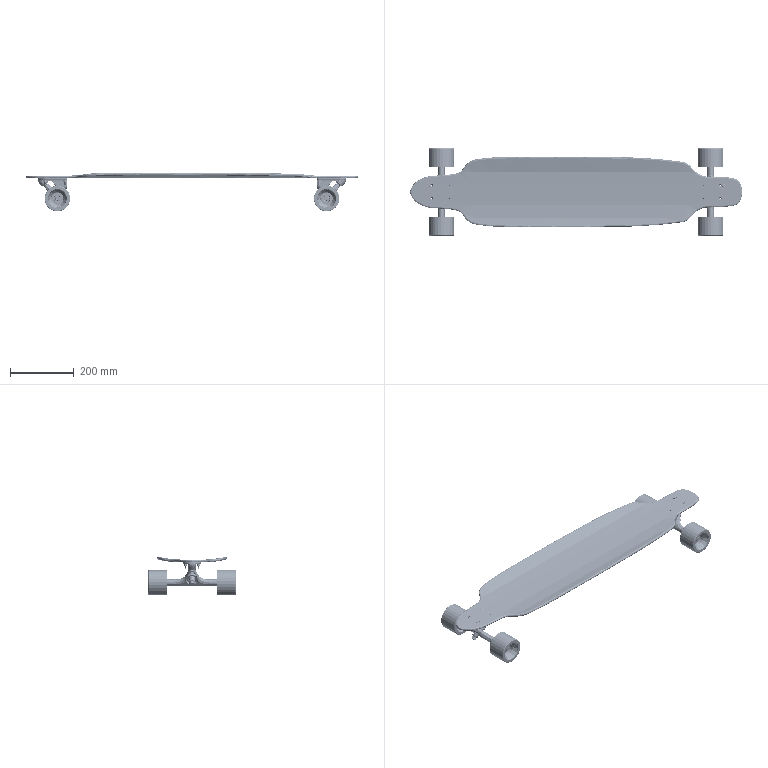Assembly | NX | mm | 63 component files | 63 solids | 1914 faces | box 1041.4 x 274 x 121.11 mm | volume 2752970 mm3 | plane 606 | cylinder 528 | cone 304 | spline 228 | torus 220 | other 20 | sphere 8 | commonest cylinder face diameters 0.26 x96 0.4 x68 0.25 x48 4 x40 6.53 x36 10 x32 5 x32 8 x20
Bill of materials:
unnamed part 1 | 7 |  | Flat circular annular ring (plain washer-like shape) with a central round through-hole and slightly rounded edges.
unnamed part 2 | 8 |  | Countersunk (flat, conical-underside) head screw with a cross-shaped recess in the head and a fully threaded straight shank.
unnamed part 3 | 4 |  | Hex nut with a cylindrical collar on one face. The collar has six radial slots and a raised inner ring around a threaded bore.
unnamed part 4 | 4 |  | Short thick-walled ring with a central bore, rounded edges and concentric annular grooves on the end face, similar in outline to a sealed ball bearing.
unnamed part 5 | 1 |  | Long, thin, flat board with a wide central section that narrows into rounded tabs at both ends. Each tab has a small group of through-holes. The board has a gentle lengthwise and crosswise curvature, similar in outline to a skateboard or longboard deck.
unnamed part 6 | 4 |  | Wide cylindrical wheel-like body with rounded outer edges, a deep recessed dished face and a small central through-bore with a stepped seat.
unnamed part 7 | 2 |  | Hollow dome-topped cylindrical cap with a thin flat flange around its open base. The base opening shows a cylindrical internal bore.
unnamed part 8 | 2 |  | Truncated cone (frustum) with a central cylindrical through-bore and rounded edges on both flat ends.
unnamed part 9 | 2 |  | Flat circular annular ring (plain washer-like shape) with a central round through-hole and slightly rounded edges.
unnamed part 10 | 1 |  | Hex nut with a cylindrical collar or shoulder on one side and a threaded central bore. The opposite face is chamfered.
unnamed part 11 | 8 |  | Hex nut with an integrated cylindrical collar on one face and a fully threaded through-bore. The hex corners are chamfered on the exposed face.
unnamed part 12 | 2 |  | Short solid cylinder (spacer or bushing-like shape) with a central cylindrical through-bore and rounded edges on both ends.
unnamed part 13 | 4 |  | Thick annular ring with a plain cylindrical outer surface, a central through bore, and concentric circular grooves on the end face near the outer and inner edges. Its overall shape looks like a sealed or shielded ball bearing.
unnamed part 14 | 2 |  | Hexagon-head bolt with a cylindrical shank. The part next to the head is unthreaded and the end portion is threaded.
unnamed part 15 | 2 |  | Long cylindrical body with stepped, smaller-diameter shafts at both ends, and both shafts end in threads. A raised curved triangular yoke in the middle holds a boss with a counterbored through hole, and a short rounded pin sticks out from the yoke's top. The overall shape looks like a skateboard-truck hanger with axle.
unnamed part 16 | 2 |  | Flat mounting plate with one rounded end and one square end, pierced by six small through holes. A U-shaped cradle or cup hangs below the plate, and it has an angled triangular side profile and a cross hole at the bottom. The overall shape looks like a skateboard-truck baseplate.
unnamed part 17 | 2 |  | Dome-shaped annular washer or bushing. One side is convex and smoothly curved, the other looks flat, and it has a central cylindrical through hole.
unnamed part 18 | 2 |  | Cup-style annular washer. One face has a stepped circular recess (counterbore) around a large central through hole, and the other side has a curved, rounded outer profile.
unnamed part 19 | 4 |  | Thin flat ring with a roughly rectangular cross-section and rounded edges. The bore is large compared with the outer diameter, so the wall is narrow.
Mates:
1. concentric | MountingNut 8 edge | MountingWasher 8 edge
2. concentric | MountingNut 7 edge | MountingWasher 7 edge
3. concentric | MountingNut 6 edge | MountingWasher 5 edge
4. concentric | MountingNut 5 edge | MountingWasher 6 edge
5. concentric | Truck 1 edge | Board1 1 arc
6. concentric | Truck 1 edge | Board1 1 arc
7. concentric | MountingWasher 4 edge | Truck 1 edge
8. concentric | MountingWasher 3 edge | Truck 1 edge
9. concentric | MountingWasher 2 edge | Truck 1 edge
10. concentric | MountingWasher 1 edge | Truck 1 edge
11. concentric | MountingNut 4 edge | MountingWasher 3 edge
12. concentric | MountingNut 3 edge | MountingWasher 1 edge
13. concentric | MountingNut 2 edge | MountingWasher 4 edge
14. concentric | MountingNut 1 edge | MountingWasher 2 edge
15. concentric | WheelsAssembly 2 edge | Truck 1 edge
16. concentric | WheelsAssembly 1 edge | Truck 1 edge